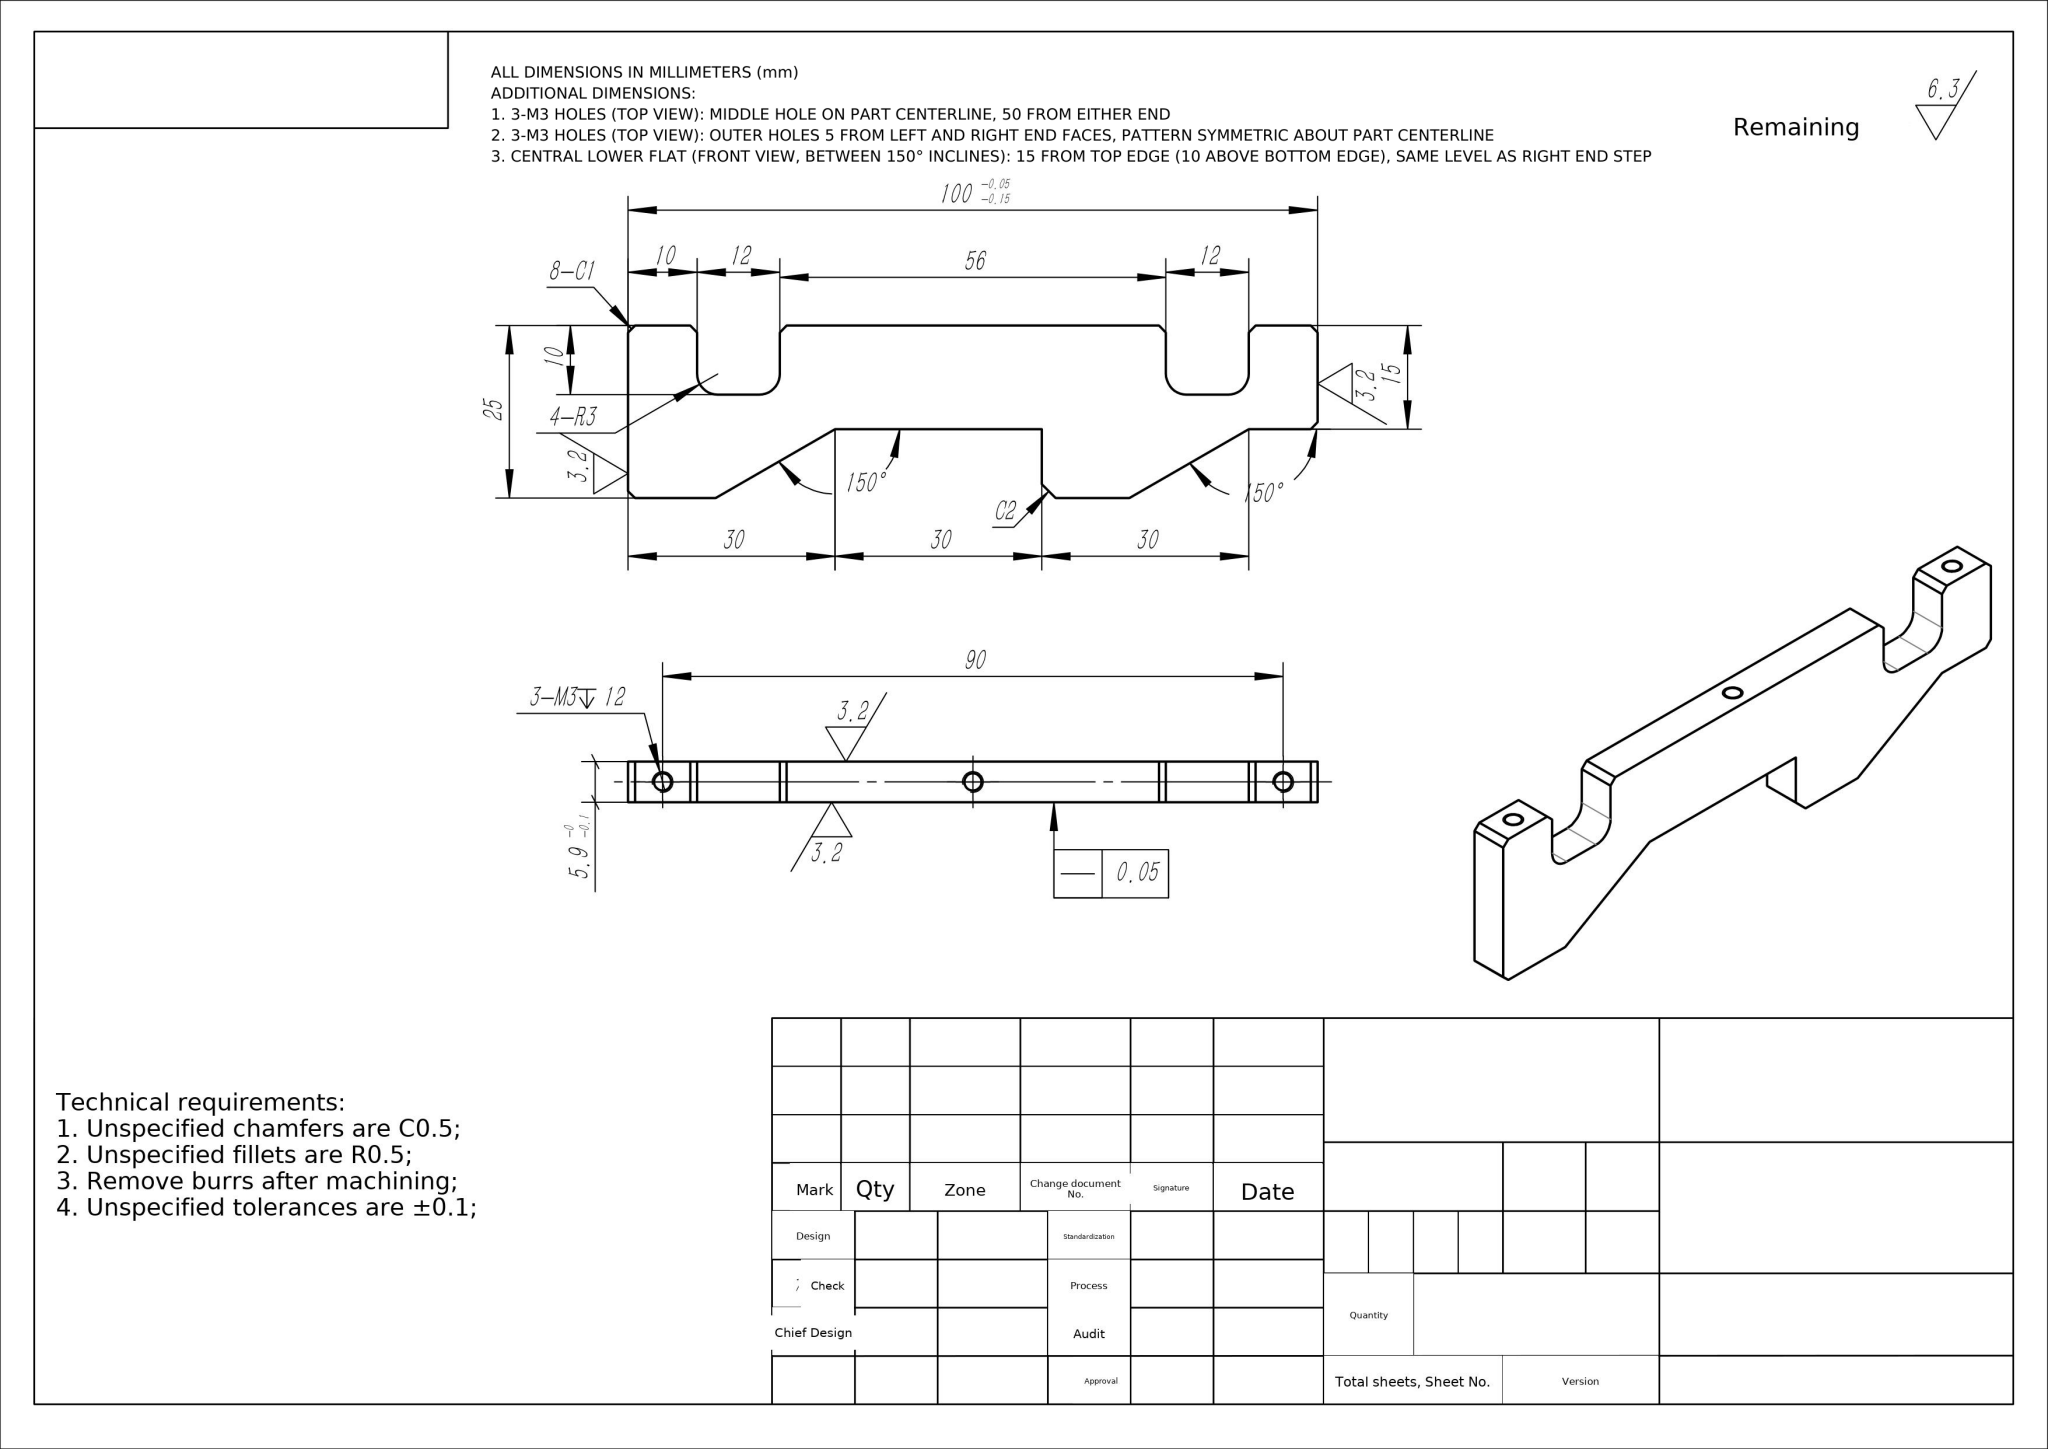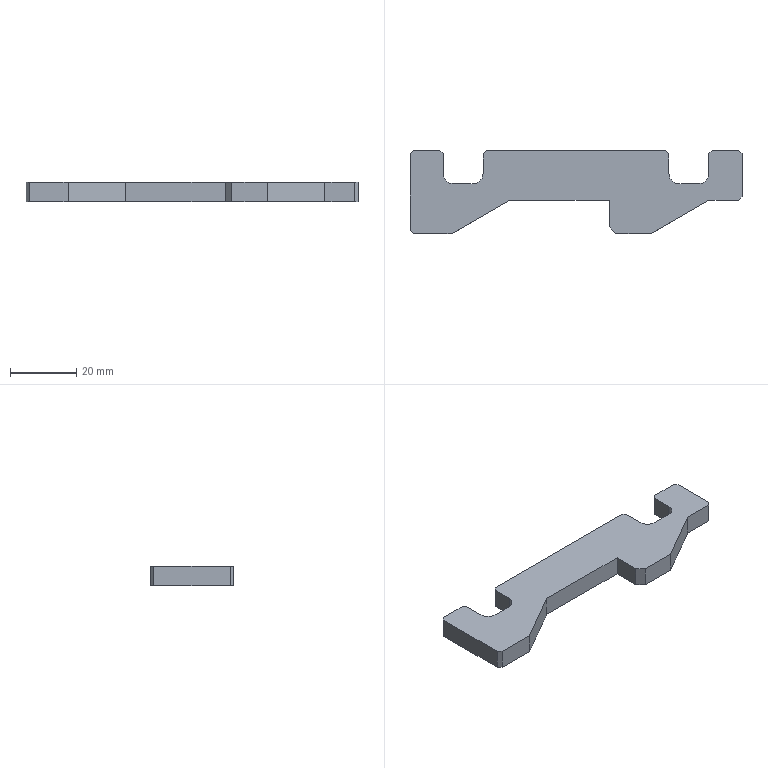Part | NX | mm | 1 solid | 45 faces | box 100 x 25 x 5.9 mm | volume 9848 mm3 | plane 29 | cylinder 10 | cone 6 | commonest cylinder face diameters 2.5 x6 6 x4